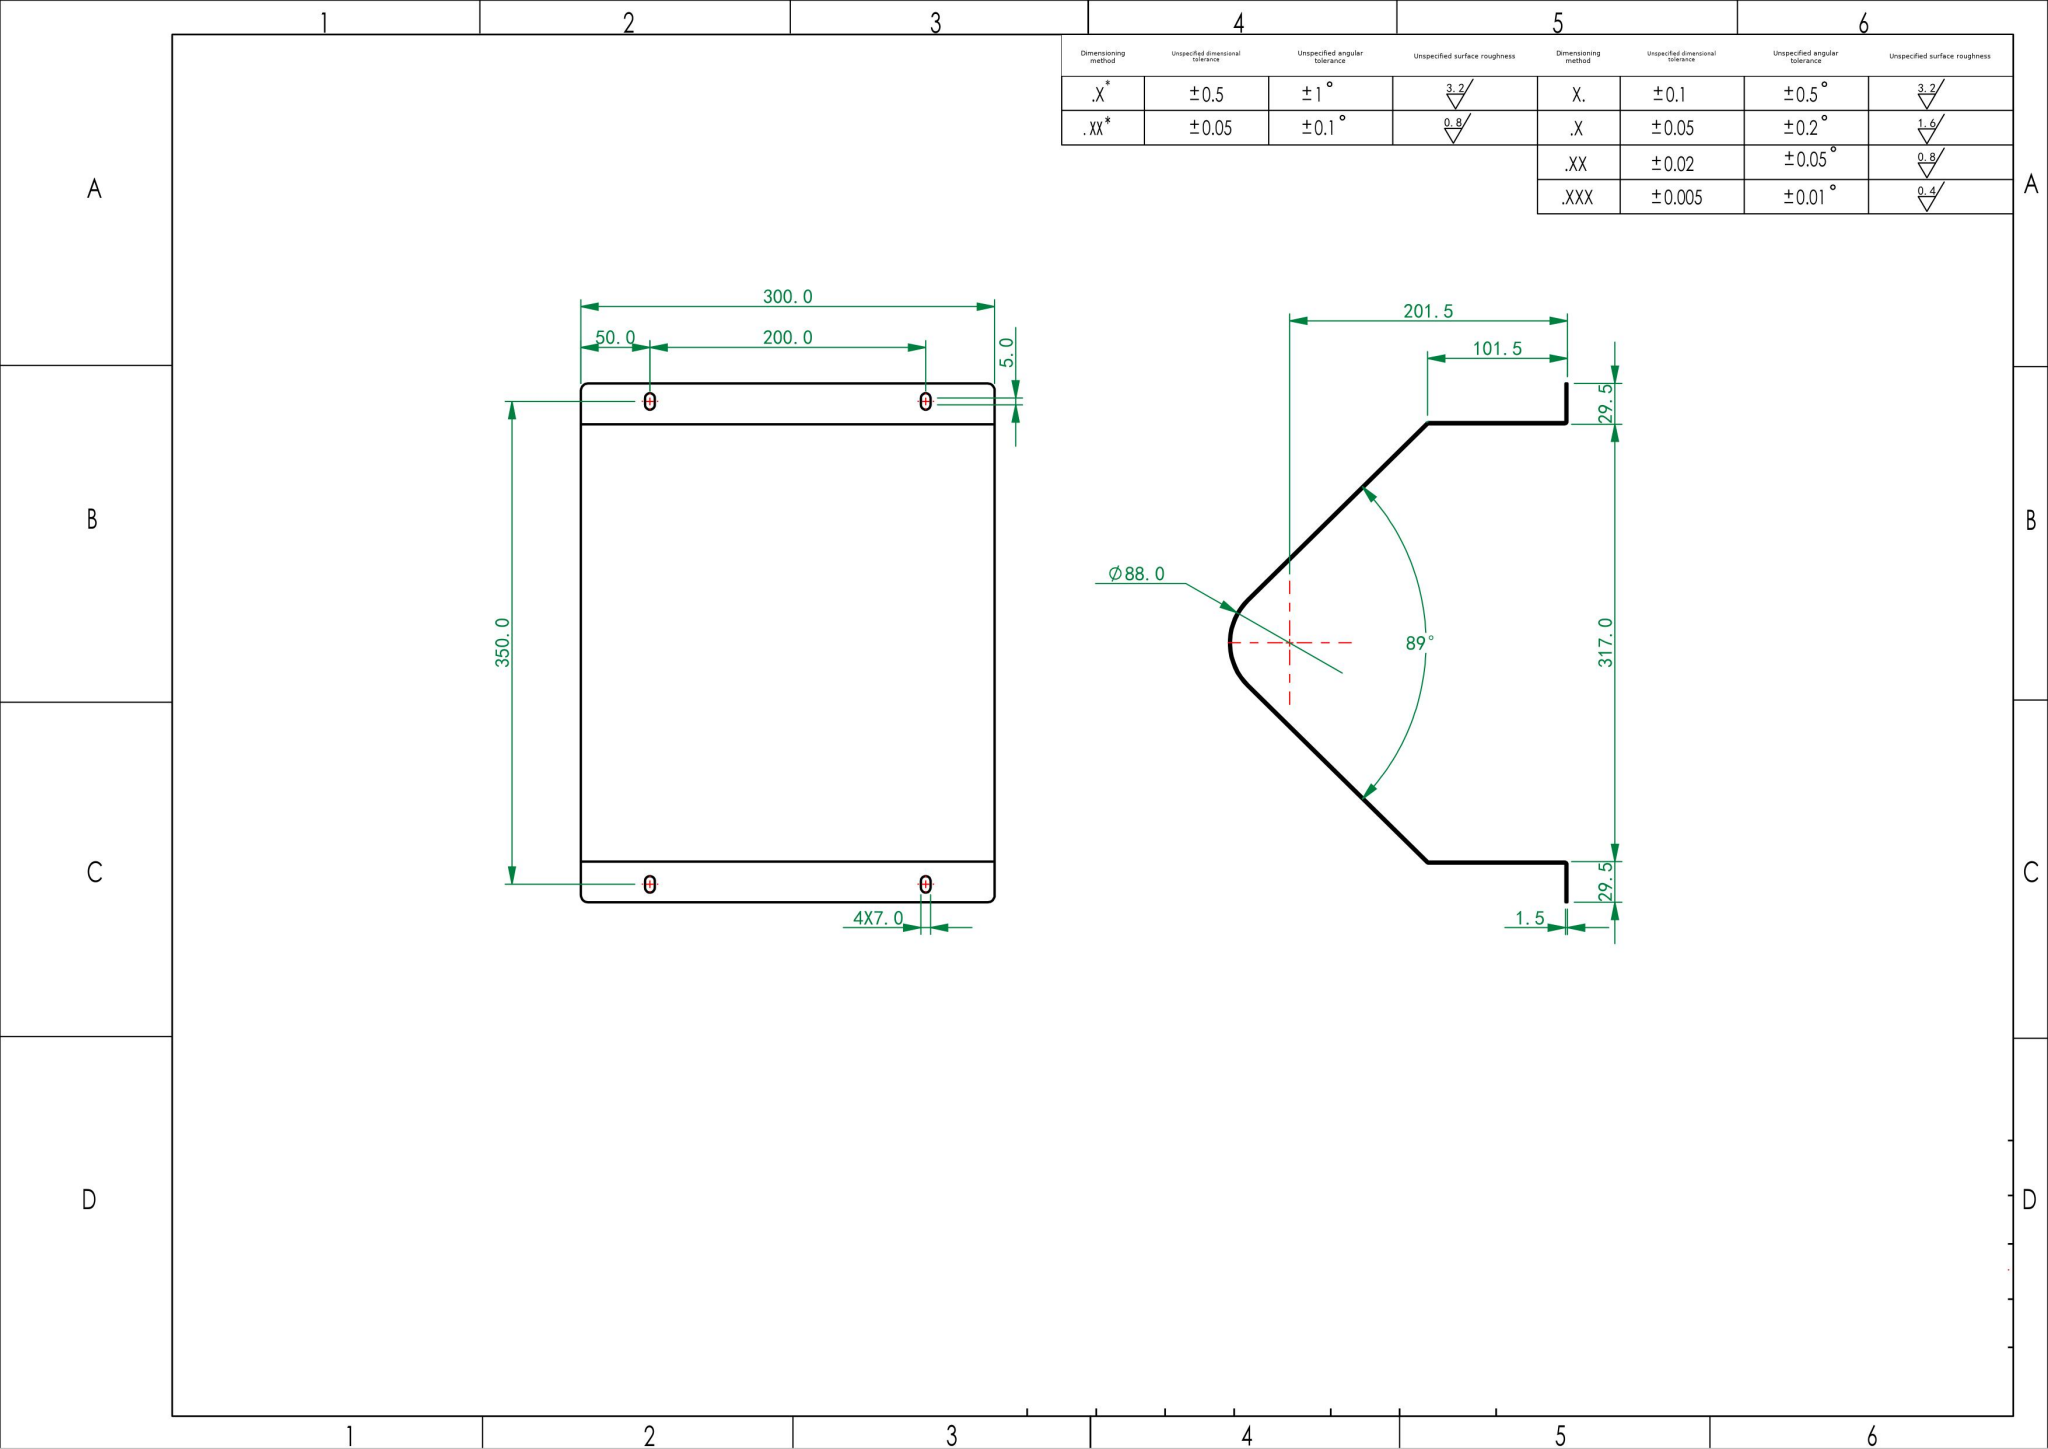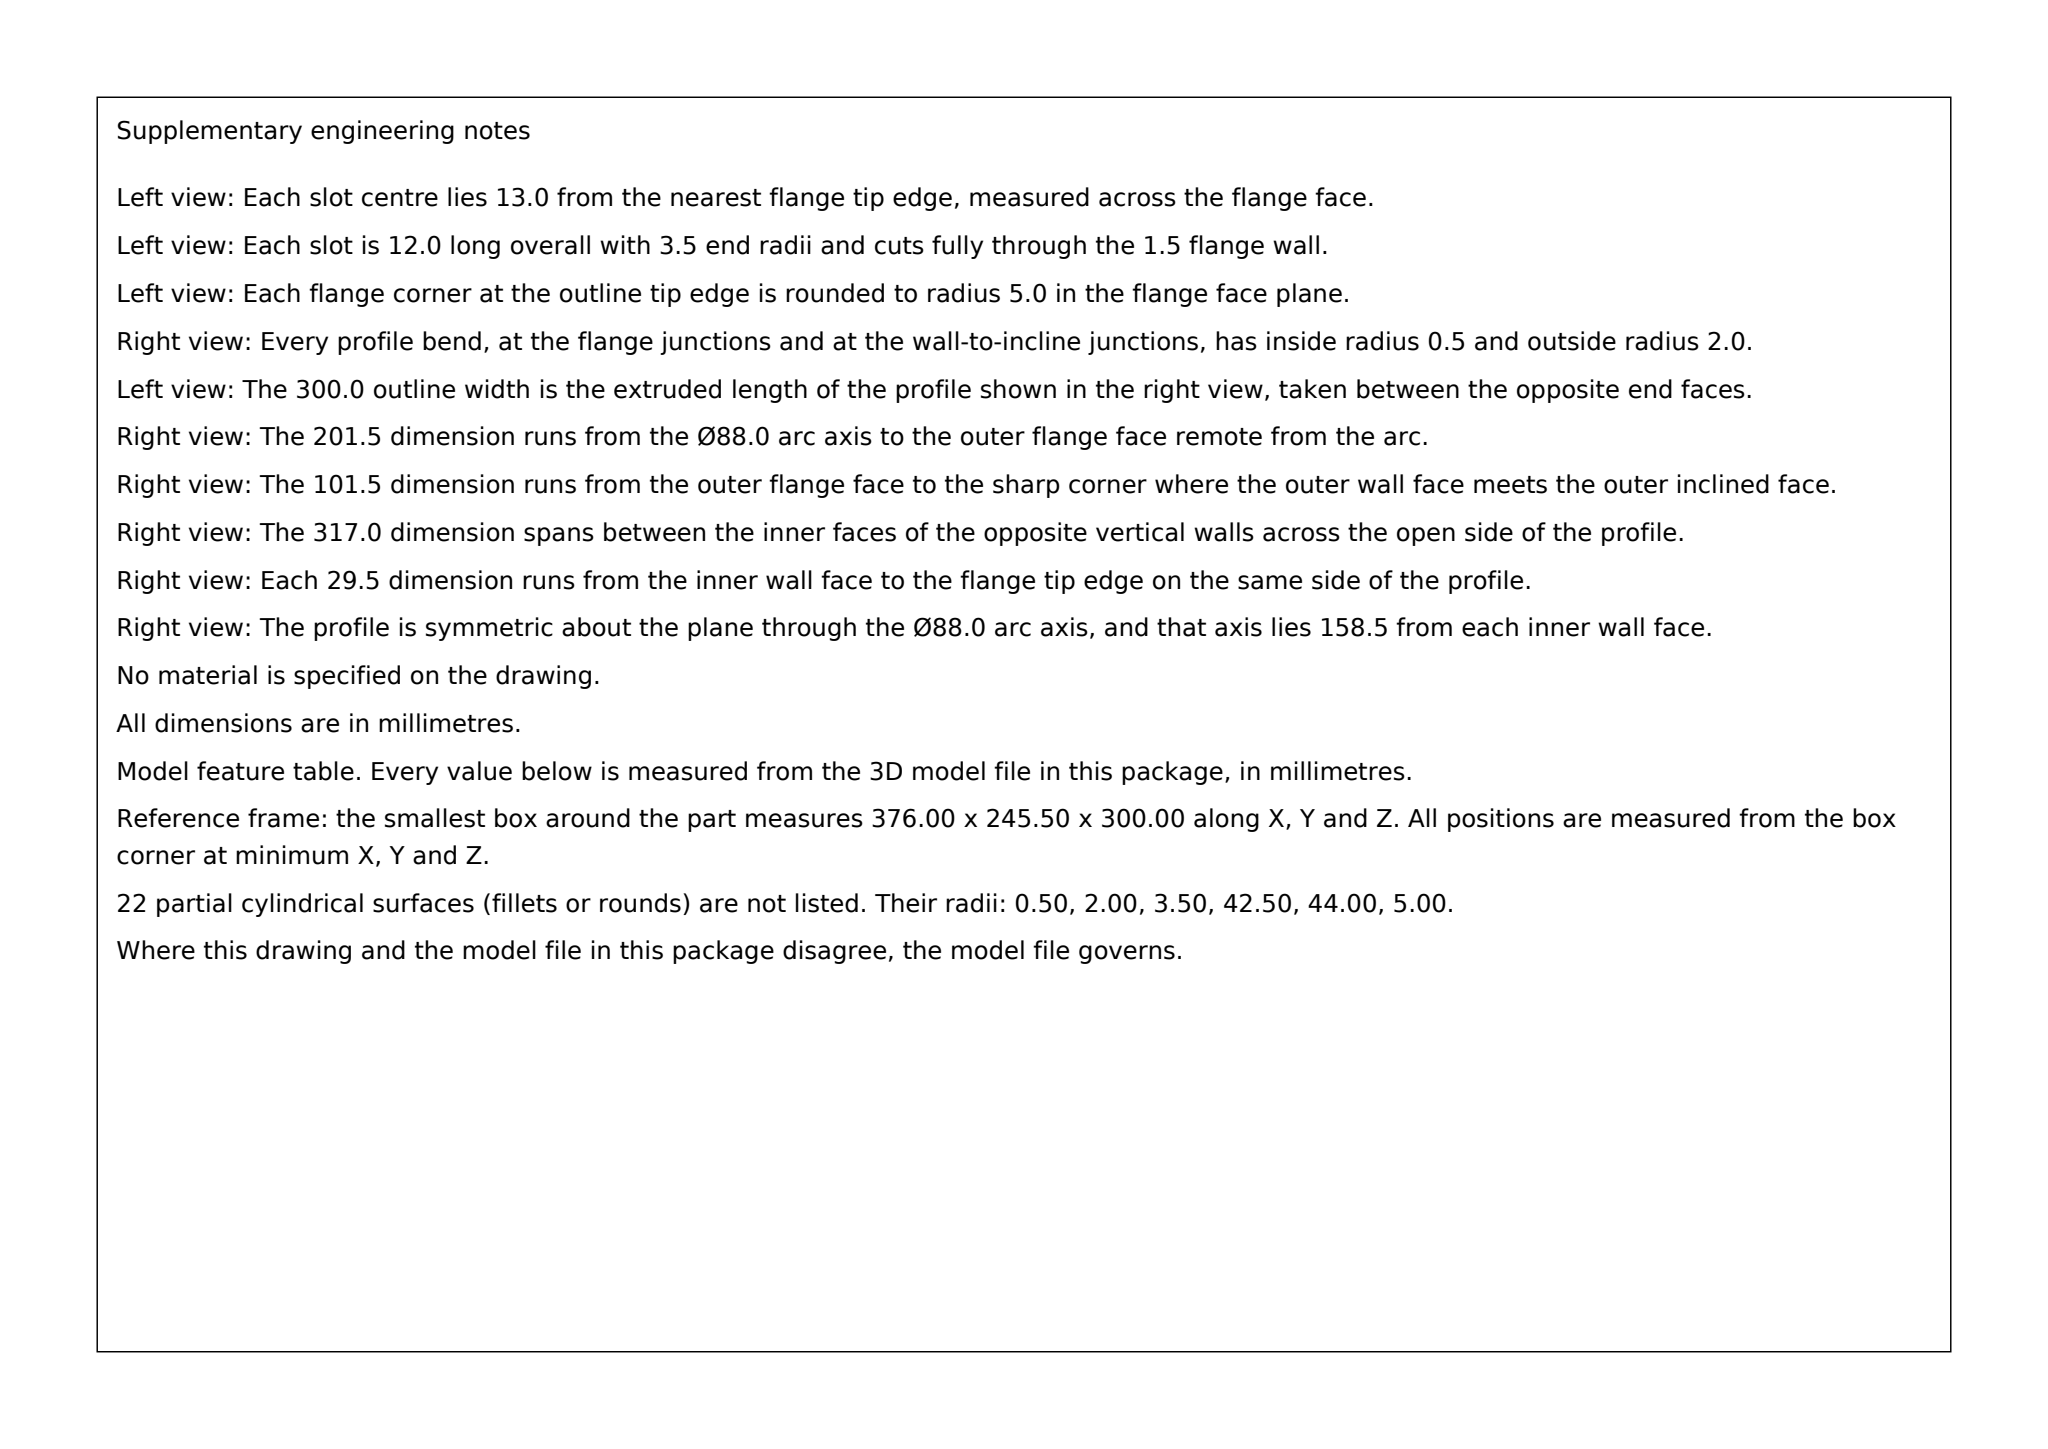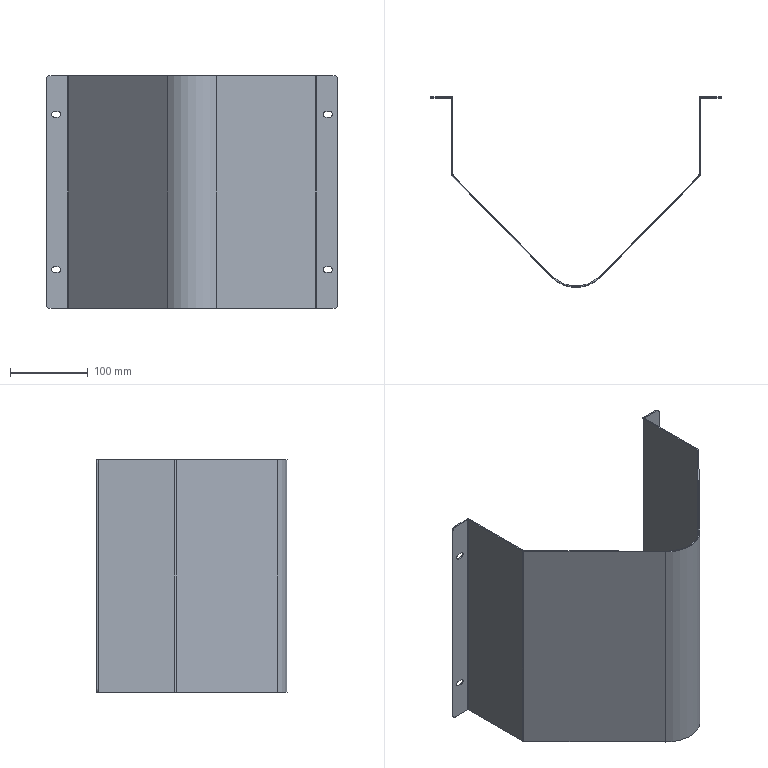Part | SolidWorks | mm | 1 solid | 70 faces | box 376 x 245.5 x 300 mm | volume 311030 mm3 | plane 44 | cylinder 26 | commonest cylinder face diameters 7 x12 1 x4 4 x4 10 x4 88 x1 85 x1
Drawing notes:
4X SLOT 7.0 WIDE X 12.0 OAL (END RADII CTRS 5.0 APART) | from the solid: 7.0 dia y-axis cyls paired at x=10.5/15.5 & 360.5/365.5 (z=50,250): 7.0+5.0 ctr spacing = 12.0 end-to-end